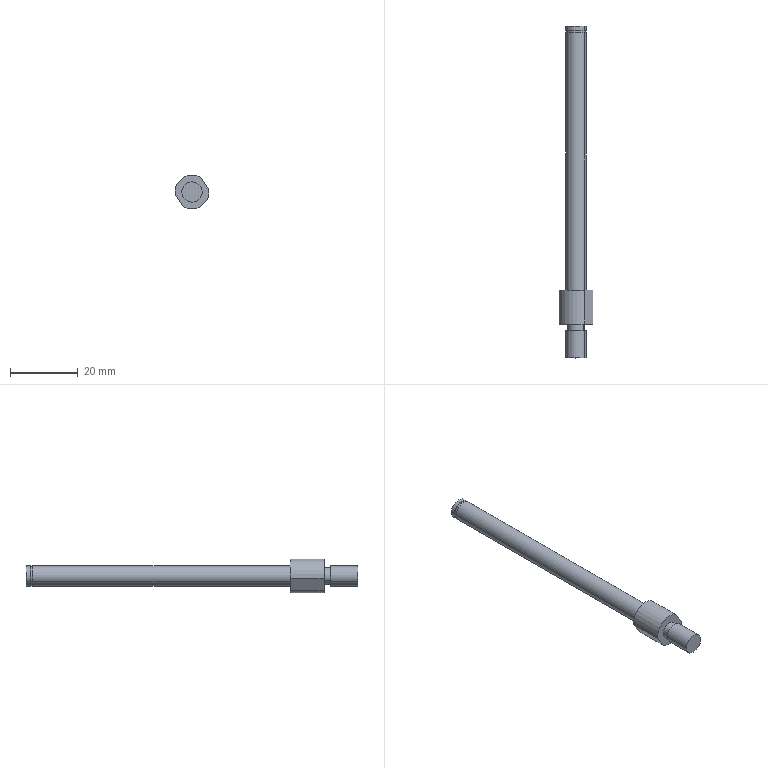Component | SolidWorks | JL001-03-06-4_JL001-03-06-001-1 | 1 solid | 21 faces | box 10 x 98 x 10 mm | volume 3224 mm3 | cylinder 12 | plane 9 | commonest cylinder face diameters 6 x6 5 x2 5.6 x2 10 x2
build123d program:
from build123d import *

# Parameters (mm, degrees)
SKETCH6_OUTSIDE_W   = 31.804
SKETCH6_OUTSIDE_H   = 31.804
SKETCH6_OUTSIDE_W_2 = 16.589
SKETCH6_OUTSIDE_H_2 = 9
CUT_EXTRUDE2_DEPTH  = 79.32


with BuildPart() as part:
    # Sketch1 → Revolve1 (revolve)
    with BuildSketch(Plane.XY, mode=Mode.PRIVATE) as revolve1_sk:
        Polygon((0, 98), (3, 98), (3, 96.8), (2.8, 96.8), (2.8, 96), (3, 96), (3, 20), (5, 20), (5, 10), (2.5, 10), (2.5, 8), (3, 8), (3, 0), (0, 0), align=None)
    revolve(revolve1_sk.sketch.rotate(Axis((0, 0, 0), (0, 1, 0)), 90), axis=Axis((0, 0, 0), (0, 1, 0)))

    # Sketch6 outside → Cut-Extrude2 (cut, through all)
    with BuildSketch(Plane(origin=(0, 20, 0), x_dir=(1, 0, 0), z_dir=(0, 1, 0))):
        Rectangle(SKETCH6_OUTSIDE_W, SKETCH6_OUTSIDE_H)
        Rectangle(SKETCH6_OUTSIDE_W_2, SKETCH6_OUTSIDE_H_2, mode=Mode.SUBTRACT)
    extrude(amount=-CUT_EXTRUDE2_DEPTH, mode=Mode.SUBTRACT)


solid = part.part

# Placed as in the assembly
solid = solid.moved(Location((-15, -47.5, 112.5), (-180, -56.842, -180)))
STEP:
#1=COLOUR_RGB('',0.7922,0.8196,0.9333);
#2=FILL_AREA_STYLE_COLOUR('',#1);
#3=FILL_AREA_STYLE('',(#2));
#4=SURFACE_STYLE_FILL_AREA(#3);
#5=SURFACE_SIDE_STYLE('',(#4));
#6=SURFACE_STYLE_USAGE(.BOTH.,#5);
#7=PRESENTATION_STYLE_ASSIGNMENT((#6));
#8=CARTESIAN_POINT('',(-0.4917,-1.555,4.494));
#9=VERTEX_POINT('',#8);
#10=CARTESIAN_POINT('',(-0.6894,-1.555,4.365));
#11=VERTEX_POINT('',#10);
#12=CARTESIAN_POINT('',(-0.5906,-1.555,4.429));
#13=DIRECTION('',(0.,-1.,0.));
#14=DIRECTION('',(0.8372,0.,0.5469));
#15=AXIS2_PLACEMENT_3D('',#12,#13,#14);
#16=CIRCLE('',#15,0.1181);
#17=EDGE_CURVE('',#9,#11,#16,.T.);
#18=ORIENTED_EDGE('',*,*,#17,.T.);
#19=CARTESIAN_POINT('',(-0.6894,-1.87,4.365));
#20=VERTEX_POINT('',#19);
#21=CARTESIAN_POINT('',(-0.6894,-1.87,4.365));
#22=DIRECTION('',(0.,-1.,0.));
#23=VECTOR('',#22,39.37);
#24=LINE('',#21,#23);
#25=EDGE_CURVE('',#11,#20,#24,.T.);
#26=ORIENTED_EDGE('',*,*,#25,.T.);
#27=CARTESIAN_POINT('',(-0.4917,-1.87,4.494));
#28=VERTEX_POINT('',#27);
#29=CARTESIAN_POINT('',(-0.5906,-1.87,4.429));
#30=DIRECTION('',(0.,-1.,0.));
#31=DIRECTION('',(0.8372,0.,0.5469));
#32=AXIS2_PLACEMENT_3D('',#29,#30,#31);
#33=CIRCLE('',#32,0.1181);
#34=EDGE_CURVE('',#28,#20,#33,.T.);
#35=ORIENTED_EDGE('',*,*,#34,.F.);
#36=CARTESIAN_POINT('',(-0.4917,-1.87,4.494));
#37=DIRECTION('',(0.,-1.,0.));
#38=VECTOR('',#37,39.37);
#39=LINE('',#36,#38);
#40=EDGE_CURVE('',#9,#28,#39,.T.);
#41=ORIENTED_EDGE('',*,*,#40,.F.);
#42=EDGE_LOOP('',(#18,#26,#35,#41));
#43=FACE_OUTER_BOUND('',#42,.T.);
#44=CARTESIAN_POINT('',(-0.5906,-1.87,4.429));
#45=DIRECTION('',(0.,-1.,0.));
#46=DIRECTION('',(0.8372,0.,0.5469));
#47=AXIS2_PLACEMENT_3D('',#44,#45,#46);
#48=CYLINDRICAL_SURFACE('',#47,0.1181);
#49=ADVANCED_FACE('',(#43),#48,.T.);
#50=CARTESIAN_POINT('',(-0.5082,-1.476,4.483));
#51=VERTEX_POINT('',#50);
#52=CARTESIAN_POINT('',(-0.6729,-1.476,4.375));
#53=VERTEX_POINT('',#52);
#54=CARTESIAN_POINT('',(-0.5906,-1.476,4.429));
#55=DIRECTION('',(0.,-1.,0.));
#56=DIRECTION('',(0.8372,0.,0.5469));
#57=AXIS2_PLACEMENT_3D('',#54,#55,#56);
#58=CIRCLE('',#57,0.09843);
#59=EDGE_CURVE('',#51,#53,#58,.T.);
#60=ORIENTED_EDGE('',*,*,#59,.T.);
#61=CARTESIAN_POINT('',(-0.6729,-1.555,4.375));
#62=VERTEX_POINT('',#61);
#63=CARTESIAN_POINT('',(-0.6729,-1.87,4.375));
#64=DIRECTION('',(0.,-1.,0.));
#65=VECTOR('',#64,39.37);
#66=LINE('',#63,#65);
#67=EDGE_CURVE('',#53,#62,#66,.T.);
#68=ORIENTED_EDGE('',*,*,#67,.T.);
#69=CARTESIAN_POINT('',(-0.5082,-1.555,4.483));
#70=VERTEX_POINT('',#69);
#71=CARTESIAN_POINT('',(-0.5906,-1.555,4.429));
#72=DIRECTION('',(0.,-1.,0.));
#73=DIRECTION('',(0.8372,0.,0.5469));
#74=AXIS2_PLACEMENT_3D('',#71,#72,#73);
#75=CIRCLE('',#74,0.09843);
#76=EDGE_CURVE('',#70,#62,#75,.T.);
#77=ORIENTED_EDGE('',*,*,#76,.F.);
#78=CARTESIAN_POINT('',(-0.5082,-1.87,4.483));
#79=DIRECTION('',(0.,-1.,0.));
#80=VECTOR('',#79,39.37);
#81=LINE('',#78,#80);
#82=EDGE_CURVE('',#51,#70,#81,.T.);
#83=ORIENTED_EDGE('',*,*,#82,.F.);
#84=EDGE_LOOP('',(#60,#68,#77,#83));
#85=FACE_OUTER_BOUND('',#84,.T.);
#86=CARTESIAN_POINT('',(-0.5906,-1.87,4.429));
#87=DIRECTION('',(0.,-1.,0.));
#88=DIRECTION('',(0.8372,0.,0.5469));
#89=AXIS2_PLACEMENT_3D('',#86,#87,#88);
#90=CYLINDRICAL_SURFACE('',#89,0.09843);
#91=ADVANCED_FACE('',(#85),#90,.T.);
#92=CARTESIAN_POINT('',(-0.4917,1.909,4.494));
#93=VERTEX_POINT('',#92);
#94=CARTESIAN_POINT('',(-0.6894,1.909,4.365));
#95=VERTEX_POINT('',#94);
#96=CARTESIAN_POINT('',(-0.5906,1.909,4.429));
#97=DIRECTION('',(0.,-1.,0.));
#98=DIRECTION('',(0.8372,0.,0.5469));
#99=AXIS2_PLACEMENT_3D('',#96,#97,#98);
#100=CIRCLE('',#99,0.1181);
#101=EDGE_CURVE('',#93,#95,#100,.T.);
#102=ORIENTED_EDGE('',*,*,#101,.T.);
#103=CARTESIAN_POINT('',(-0.6894,-1.083,4.365));
#104=VERTEX_POINT('',#103);
#105=CARTESIAN_POINT('',(-0.6894,-1.87,4.365));
#106=DIRECTION('',(0.,-1.,0.));
#107=VECTOR('',#106,39.37);
#108=LINE('',#105,#107);
#109=EDGE_CURVE('',#95,#104,#108,.T.);
#110=ORIENTED_EDGE('',*,*,#109,.T.);
#111=CARTESIAN_POINT('',(-0.4917,-1.083,4.494));
#112=VERTEX_POINT('',#111);
#113=CARTESIAN_POINT('',(-0.5906,-1.083,4.429));
#114=DIRECTION('',(0.,-1.,0.));
#115=DIRECTION('',(0.8372,0.,0.5469));
#116=AXIS2_PLACEMENT_3D('',#113,#114,#115);
#117=CIRCLE('',#116,0.1181);
#118=EDGE_CURVE('',#112,#104,#117,.T.);
#119=ORIENTED_EDGE('',*,*,#118,.F.);
#120=CARTESIAN_POINT('',(-0.4917,-1.87,4.494));
#121=DIRECTION('',(0.,-1.,0.));
#122=VECTOR('',#121,39.37);
#123=LINE('',#120,#122);
#124=EDGE_CURVE('',#93,#112,#123,.T.);
#125=ORIENTED_EDGE('',*,*,#124,.F.);
#126=EDGE_LOOP('',(#102,#110,#119,#125));
#127=FACE_OUTER_BOUND('',#126,.T.);
#128=CARTESIAN_POINT('',(-0.5906,-1.87,4.429));
#129=DIRECTION('',(0.,-1.,0.));
#130=DIRECTION('',(0.8372,0.,0.5469));
#131=AXIS2_PLACEMENT_3D('',#128,#129,#130);
#132=CYLINDRICAL_SURFACE('',#131,0.1181);
#133=ADVANCED_FACE('',(#127),#132,.T.);
#134=CARTESIAN_POINT('',(-0.4983,1.941,4.489));
#135=VERTEX_POINT('',#134);
#136=CARTESIAN_POINT('',(-0.6828,1.941,4.369));
#137=VERTEX_POINT('',#136);
#138=CARTESIAN_POINT('',(-0.5906,1.941,4.429));
#139=DIRECTION('',(0.,-1.,0.));
#140=DIRECTION('',(0.8372,0.,0.5469));
#141=AXIS2_PLACEMENT_3D('',#138,#139,#140);
#142=CIRCLE('',#141,0.1102);
#143=EDGE_CURVE('',#135,#137,#142,.T.);
#144=ORIENTED_EDGE('',*,*,#143,.T.);
#145=CARTESIAN_POINT('',(-0.6828,1.909,4.369));
#146=VERTEX_POINT('',#145);
#147=CARTESIAN_POINT('',(-0.6828,-1.87,4.369));
#148=DIRECTION('',(0.,-1.,0.));
#149=VECTOR('',#148,39.37);
#150=LINE('',#147,#149);
#151=EDGE_CURVE('',#137,#146,#150,.T.);
#152=ORIENTED_EDGE('',*,*,#151,.T.);
#153=CARTESIAN_POINT('',(-0.4983,1.909,4.489));
#154=VERTEX_POINT('',#153);
#155=CARTESIAN_POINT('',(-0.5906,1.909,4.429));
#156=DIRECTION('',(0.,-1.,0.));
#157=DIRECTION('',(0.8372,0.,0.5469));
#158=AXIS2_PLACEMENT_3D('',#155,#156,#157);
#159=CIRCLE('',#158,0.1102);
#160=EDGE_CURVE('',#154,#146,#159,.T.);
#161=ORIENTED_EDGE('',*,*,#160,.F.);
#162=CARTESIAN_POINT('',(-0.4983,-1.87,4.489));
#163=DIRECTION('',(0.,-1.,0.));
#164=VECTOR('',#163,39.37);
#165=LINE('',#162,#164);
#166=EDGE_CURVE('',#135,#154,#165,.T.);
#167=ORIENTED_EDGE('',*,*,#166,.F.);
#168=EDGE_LOOP('',(#144,#152,#161,#167));
#169=FACE_OUTER_BOUND('',#168,.T.);
#170=CARTESIAN_POINT('',(-0.5906,-1.87,4.429));
#171=DIRECTION('',(0.,-1.,0.));
#172=DIRECTION('',(0.8372,0.,0.5469));
#173=AXIS2_PLACEMENT_3D('',#170,#171,#172);
#174=CYLINDRICAL_SURFACE('',#173,0.1102);
#175=ADVANCED_FACE('',(#169),#174,.T.);
#176=CARTESIAN_POINT('',(-0.4917,1.988,4.494));
#177=VERTEX_POINT('',#176);
#178=CARTESIAN_POINT('',(-0.6894,1.988,4.365));
#179=VERTEX_POINT('',#178);
#180=CARTESIAN_POINT('',(-0.5906,1.988,4.429));
#181=DIRECTION('',(0.,-1.,0.));
#182=DIRECTION('',(0.8372,0.,0.5469));
#183=AXIS2_PLACEMENT_3D('',#180,#181,#182);
#184=CIRCLE('',#183,0.1181);
#185=EDGE_CURVE('',#177,#179,#184,.T.);
#186=ORIENTED_EDGE('',*,*,#185,.T.);
#187=CARTESIAN_POINT('',(-0.6894,1.941,4.365));
#188=VERTEX_POINT('',#187);
#189=CARTESIAN_POINT('',(-0.6894,-1.87,4.365));
#190=DIRECTION('',(0.,-1.,0.));
#191=VECTOR('',#190,39.37);
#192=LINE('',#189,#191);
#193=EDGE_CURVE('',#179,#188,#192,.T.);
#194=ORIENTED_EDGE('',*,*,#193,.T.);
#195=CARTESIAN_POINT('',(-0.4917,1.941,4.494));
#196=VERTEX_POINT('',#195);
#197=CARTESIAN_POINT('',(-0.5906,1.941,4.429));
#198=DIRECTION('',(0.,-1.,0.));
#199=DIRECTION('',(0.8372,0.,0.5469));
#200=AXIS2_PLACEMENT_3D('',#197,#198,#199);
#201=CIRCLE('',#200,0.1181);
#202=EDGE_CURVE('',#196,#188,#201,.T.);
#203=ORIENTED_EDGE('',*,*,#202,.F.);
#204=CARTESIAN_POINT('',(-0.4917,-1.87,4.494));
#205=DIRECTION('',(0.,-1.,0.));
#206=VECTOR('',#205,39.37);
#207=LINE('',#204,#206);
#208=EDGE_CURVE('',#177,#196,#207,.T.);
#209=ORIENTED_EDGE('',*,*,#208,.F.);
#210=EDGE_LOOP('',(#186,#194,#203,#209));
#211=FACE_OUTER_BOUND('',#210,.T.);
#212=CARTESIAN_POINT('',(-0.5906,-1.87,4.429));
#213=DIRECTION('',(0.,-1.,0.));
#214=DIRECTION('',(0.8372,0.,0.5469));
#215=AXIS2_PLACEMENT_3D('',#212,#213,#214);
#216=CYLINDRICAL_SURFACE('',#215,0.1181);
#217=ADVANCED_FACE('',(#211),#216,.T.);
#218=ORIENTED_EDGE('',*,*,#118,.T.);
#219=CARTESIAN_POINT('',(-0.5906,-1.083,4.429));
#220=DIRECTION('',(0.,-1.,0.));
#221=DIRECTION('',(0.8372,0.,0.5469));
#222=AXIS2_PLACEMENT_3D('',#219,#220,#221);
#223=CIRCLE('',#222,0.1181);
#224=EDGE_CURVE('',#104,#112,#223,.T.);
#225=ORIENTED_EDGE('',*,*,#224,.T.);
#226=EDGE_LOOP('',(#218,#225));
#227=FACE_BOUND('',#226,.T.);
#228=CARTESIAN_POINT('',(-0.6919,-1.083,4.26));
#229=VERTEX_POINT('',#228);
#230=CARTESIAN_POINT('',(-0.3953,-1.083,4.454));
#231=VERTEX_POINT('',#230);
#232=CARTESIAN_POINT('',(-0.5906,-1.083,4.429));
#233=DIRECTION('',(0.,-1.,0.));
#234=DIRECTION('',(0.8372,0.,0.5469));
#235=AXIS2_PLACEMENT_3D('',#232,#233,#234);
#236=CIRCLE('',#235,0.1969);
#237=EDGE_CURVE('',#229,#231,#236,.T.);
#238=ORIENTED_EDGE('',*,*,#237,.F.);
#239=CARTESIAN_POINT('',(-0.7858,-1.083,4.404));
#240=VERTEX_POINT('',#239);
#241=CARTESIAN_POINT('',(-0.5603,-1.083,4.059));
#242=DIRECTION('',(-0.5469,0.,0.8372));
#243=VECTOR('',#242,39.37);
#244=LINE('',#241,#243);
#245=EDGE_CURVE('',#229,#240,#244,.T.);
#246=ORIENTED_EDGE('',*,*,#245,.T.);
#247=CARTESIAN_POINT('',(-0.4892,-1.083,4.598));
#248=VERTEX_POINT('',#247);
#249=CARTESIAN_POINT('',(-0.5906,-1.083,4.429));
#250=DIRECTION('',(0.,-1.,0.));
#251=DIRECTION('',(0.8372,0.,0.5469));
#252=AXIS2_PLACEMENT_3D('',#249,#250,#251);
#253=CIRCLE('',#252,0.1969);
#254=EDGE_CURVE('',#248,#240,#253,.T.);
#255=ORIENTED_EDGE('',*,*,#254,.F.);
#256=CARTESIAN_POINT('',(-0.2636,-1.083,4.253));
#257=DIRECTION('',(0.5469,0.,-0.8372));
#258=VECTOR('',#257,39.37);
#259=LINE('',#256,#258);
#260=EDGE_CURVE('',#248,#231,#259,.T.);
#261=ORIENTED_EDGE('',*,*,#260,.T.);
#262=EDGE_LOOP('',(#238,#246,#255,#261));
#263=FACE_OUTER_BOUND('',#262,.T.);
#264=CARTESIAN_POINT('',(-0.6552,-1.083,4.528));
#265=DIRECTION('',(0.,1.,0.));
#266=DIRECTION('',(-0.8372,0.,-0.5469));
#267=AXIS2_PLACEMENT_3D('',#264,#265,#266);
#268=PLANE('',#267);
#269=ADVANCED_FACE('',(#227,#263),#268,.T.);
#270=CARTESIAN_POINT('',(-0.6919,-1.476,4.26));
#271=VERTEX_POINT('',#270);
#272=CARTESIAN_POINT('',(-0.3953,-1.476,4.454));
#273=VERTEX_POINT('',#272);
#274=CARTESIAN_POINT('',(-0.5906,-1.476,4.429));
#275=DIRECTION('',(0.,-1.,0.));
#276=DIRECTION('',(0.8372,0.,0.5469));
#277=AXIS2_PLACEMENT_3D('',#274,#275,#276);
#278=CIRCLE('',#277,0.1969);
#279=EDGE_CURVE('',#271,#273,#278,.T.);
#280=ORIENTED_EDGE('',*,*,#279,.F.);
#281=CARTESIAN_POINT('',(-0.6919,-1.87,4.26));
#282=DIRECTION('',(0.,1.,0.));
#283=VECTOR('',#282,39.37);
#284=LINE('',#281,#283);
#285=EDGE_CURVE('',#271,#229,#284,.T.);
#286=ORIENTED_EDGE('',*,*,#285,.T.);
#287=ORIENTED_EDGE('',*,*,#237,.T.);
#288=CARTESIAN_POINT('',(-0.3953,-1.87,4.454));
#289=DIRECTION('',(0.,-1.,0.));
#290=VECTOR('',#289,39.37);
#291=LINE('',#288,#290);
#292=EDGE_CURVE('',#231,#273,#291,.T.);
#293=ORIENTED_EDGE('',*,*,#292,.T.);
#294=EDGE_LOOP('',(#280,#286,#287,#293));
#295=FACE_OUTER_BOUND('',#294,.T.);
#296=CARTESIAN_POINT('',(-0.5906,-1.87,4.429));
#297=DIRECTION('',(0.,-1.,0.));
#298=DIRECTION('',(0.8372,0.,0.5469));
#299=AXIS2_PLACEMENT_3D('',#296,#297,#298);
#300=CYLINDRICAL_SURFACE('',#299,0.1969);
#301=ADVANCED_FACE('',(#295),#300,.T.);
#302=ORIENTED_EDGE('',*,*,#254,.T.);
#303=CARTESIAN_POINT('',(-0.7858,-1.476,4.404));
#304=VERTEX_POINT('',#303);
#305=CARTESIAN_POINT('',(-0.7858,-1.87,4.404));
#306=DIRECTION('',(0.,-1.,0.));
#307=VECTOR('',#306,39.37);
#308=LINE('',#305,#307);
#309=EDGE_CURVE('',#240,#304,#308,.T.);
#310=ORIENTED_EDGE('',*,*,#309,.T.);
#311=CARTESIAN_POINT('',(-0.4892,-1.476,4.598));
#312=VERTEX_POINT('',#311);
#313=CARTESIAN_POINT('',(-0.5906,-1.476,4.429));
#314=DIRECTION('',(0.,-1.,0.));
#315=DIRECTION('',(0.8372,0.,0.5469));
#316=AXIS2_PLACEMENT_3D('',#313,#314,#315);
#317=CIRCLE('',#316,0.1969);
#318=EDGE_CURVE('',#312,#304,#317,.T.);
#319=ORIENTED_EDGE('',*,*,#318,.F.);
#320=CARTESIAN_POINT('',(-0.4892,-1.87,4.598));
#321=DIRECTION('',(0.,1.,0.));
#322=VECTOR('',#321,39.37);
#323=LINE('',#320,#322);
#324=EDGE_CURVE('',#312,#248,#323,.T.);
#325=ORIENTED_EDGE('',*,*,#324,.T.);
#326=EDGE_LOOP('',(#302,#310,#319,#325));
#327=FACE_OUTER_BOUND('',#326,.T.);
#328=CARTESIAN_POINT('',(-0.5906,-1.87,4.429));
#329=DIRECTION('',(0.,-1.,0.));
#330=DIRECTION('',(0.8372,0.,0.5469));
#331=AXIS2_PLACEMENT_3D('',#328,#329,#330);
#332=CYLINDRICAL_SURFACE('',#331,0.1969);
#333=ADVANCED_FACE('',(#327),#332,.T.);
#334=ORIENTED_EDGE('',*,*,#59,.F.);
#335=CARTESIAN_POINT('',(-0.5906,-1.476,4.429));
#336=DIRECTION('',(0.,-1.,0.));
#337=DIRECTION('',(0.8372,0.,0.5469));
#338=AXIS2_PLACEMENT_3D('',#335,#336,#337);
#339=CIRCLE('',#338,0.09843);
#340=EDGE_CURVE('',#53,#51,#339,.T.);
#341=ORIENTED_EDGE('',*,*,#340,.F.);
#342=EDGE_LOOP('',(#334,#341));
#343=FACE_BOUND('',#342,.T.);
#344=ORIENTED_EDGE('',*,*,#318,.T.);
#345=CARTESIAN_POINT('',(-0.8465,-1.476,4.497));
#346=DIRECTION('',(0.5469,0.,-0.8372));
#347=VECTOR('',#346,39.37);
#348=LINE('',#345,#347);
#349=EDGE_CURVE('',#304,#271,#348,.T.);
#350=ORIENTED_EDGE('',*,*,#349,.T.);
#351=ORIENTED_EDGE('',*,*,#279,.T.);
#352=CARTESIAN_POINT('',(-0.5499,-1.476,4.691));
#353=DIRECTION('',(-0.5469,0.,0.8372));
#354=VECTOR('',#353,39.37);
#355=LINE('',#352,#354);
#356=EDGE_CURVE('',#273,#312,#355,.T.);
#357=ORIENTED_EDGE('',*,*,#356,.T.);
#358=EDGE_LOOP('',(#344,#350,#351,#357));
#359=FACE_OUTER_BOUND('',#358,.T.);
#360=CARTESIAN_POINT('',(-0.6982,-1.476,4.594));
#361=DIRECTION('',(0.,-1.,0.));
#362=DIRECTION('',(0.8372,0.,0.5469));
#363=AXIS2_PLACEMENT_3D('',#360,#361,#362);
#364=PLANE('',#363);
#365=ADVANCED_FACE('',(#343,#359),#364,.T.);
#366=ORIENTED_EDGE('',*,*,#185,.F.);
#367=CARTESIAN_POINT('',(-0.5906,1.988,4.429));
#368=DIRECTION('',(0.,-1.,0.));
#369=DIRECTION('',(0.8372,0.,0.5469));
#370=AXIS2_PLACEMENT_3D('',#367,#368,#369);
#371=CIRCLE('',#370,0.1181);
#372=EDGE_CURVE('',#179,#177,#371,.T.);
#373=ORIENTED_EDGE('',*,*,#372,.F.);
#374=EDGE_LOOP('',(#366,#373));
#375=FACE_OUTER_BOUND('',#374,.T.);
#376=CARTESIAN_POINT('',(-0.5906,1.988,4.429));
#377=DIRECTION('',(0.,1.,0.));
#378=DIRECTION('',(-0.8372,0.,-0.5469));
#379=AXIS2_PLACEMENT_3D('',#376,#377,#378);
#380=PLANE('',#379);
#381=ADVANCED_FACE('',(#375),#380,.T.);
#382=ORIENTED_EDGE('',*,*,#193,.F.);
#383=ORIENTED_EDGE('',*,*,#372,.T.);
#384=ORIENTED_EDGE('',*,*,#208,.T.);
#385=CARTESIAN_POINT('',(-0.5906,1.941,4.429));
#386=DIRECTION('',(0.,-1.,0.));
#387=DIRECTION('',(0.8372,0.,0.5469));
#388=AXIS2_PLACEMENT_3D('',#385,#386,#387);
#389=CIRCLE('',#388,0.1181);
#390=EDGE_CURVE('',#188,#196,#389,.T.);
#391=ORIENTED_EDGE('',*,*,#390,.F.);
#392=EDGE_LOOP('',(#382,#383,#384,#391));
#393=FACE_OUTER_BOUND('',#392,.T.);
#394=CARTESIAN_POINT('',(-0.5906,-1.87,4.429));
#395=DIRECTION('',(0.,-1.,0.));
#396=DIRECTION('',(0.8372,0.,0.5469));
#397=AXIS2_PLACEMENT_3D('',#394,#395,#396);
#398=CYLINDRICAL_SURFACE('',#397,0.1181);
#399=ADVANCED_FACE('',(#393),#398,.T.);
#400=ORIENTED_EDGE('',*,*,#202,.T.);
#401=ORIENTED_EDGE('',*,*,#390,.T.);
#402=EDGE_LOOP('',(#400,#401));
#403=FACE_OUTER_BOUND('',#402,.T.);
#404=ORIENTED_EDGE('',*,*,#143,.F.);
#405=CARTESIAN_POINT('',(-0.5906,1.941,4.429));
#406=DIRECTION('',(0.,-1.,0.));
#407=DIRECTION('',(0.8372,0.,0.5469));
#408=AXIS2_PLACEMENT_3D('',#405,#406,#407);
#409=CIRCLE('',#408,0.1102);
#410=EDGE_CURVE('',#137,#135,#409,.T.);
#411=ORIENTED_EDGE('',*,*,#410,.F.);
#412=EDGE_LOOP('',(#404,#411));
#413=FACE_BOUND('',#412,.T.);
#414=CARTESIAN_POINT('',(-0.6552,1.941,4.528));
#415=DIRECTION('',(0.,-1.,0.));
#416=DIRECTION('',(0.8372,0.,0.5469));
#417=AXIS2_PLACEMENT_3D('',#414,#415,#416);
#418=PLANE('',#417);
#419=ADVANCED_FACE('',(#403,#413),#418,.T.);
#420=ORIENTED_EDGE('',*,*,#151,.F.);
#421=ORIENTED_EDGE('',*,*,#410,.T.);
#422=ORIENTED_EDGE('',*,*,#166,.T.);
#423=CARTESIAN_POINT('',(-0.5906,1.909,4.429));
#424=DIRECTION('',(0.,-1.,0.));
#425=DIRECTION('',(0.8372,0.,0.5469));
#426=AXIS2_PLACEMENT_3D('',#423,#424,#425);
#427=CIRCLE('',#426,0.1102);
#428=EDGE_CURVE('',#146,#154,#427,.T.);
#429=ORIENTED_EDGE('',*,*,#428,.F.);
#430=EDGE_LOOP('',(#420,#421,#422,#429));
#431=FACE_OUTER_BOUND('',#430,.T.);
#432=CARTESIAN_POINT('',(-0.5906,-1.87,4.429));
#433=DIRECTION('',(0.,-1.,0.));
#434=DIRECTION('',(0.8372,0.,0.5469));
#435=AXIS2_PLACEMENT_3D('',#432,#433,#434);
#436=CYLINDRICAL_SURFACE('',#435,0.1102);
#437=ADVANCED_FACE('',(#431),#436,.T.);
#438=ORIENTED_EDGE('',*,*,#160,.T.);
#439=ORIENTED_EDGE('',*,*,#428,.T.);
#440=EDGE_LOOP('',(#438,#439));
#441=FACE_BOUND('',#440,.T.);
#442=ORIENTED_EDGE('',*,*,#101,.F.);
#443=CARTESIAN_POINT('',(-0.5906,1.909,4.429));
#444=DIRECTION('',(0.,-1.,0.));
#445=DIRECTION('',(0.8372,0.,0.5469));
#446=AXIS2_PLACEMENT_3D('',#443,#444,#445);
#447=CIRCLE('',#446,0.1181);
#448=EDGE_CURVE('',#95,#93,#447,.T.);
#449=ORIENTED_EDGE('',*,*,#448,.F.);
#450=EDGE_LOOP('',(#442,#449));
#451=FACE_OUTER_BOUND('',#450,.T.);
#452=CARTESIAN_POINT('',(-0.6508,1.909,4.521));
#453=DIRECTION('',(0.,1.,0.));
#454=DIRECTION('',(-0.8372,0.,-0.5469));
#455=AXIS2_PLACEMENT_3D('',#452,#453,#454);
#456=PLANE('',#455);
#457=ADVANCED_FACE('',(#441,#451),#456,.T.);
#458=ORIENTED_EDGE('',*,*,#109,.F.);
#459=ORIENTED_EDGE('',*,*,#448,.T.);
#460=ORIENTED_EDGE('',*,*,#124,.T.);
#461=ORIENTED_EDGE('',*,*,#224,.F.);
#462=EDGE_LOOP('',(#458,#459,#460,#461));
#463=FACE_OUTER_BOUND('',#462,.T.);
#464=CARTESIAN_POINT('',(-0.5906,-1.87,4.429));
#465=DIRECTION('',(0.,-1.,0.));
#466=DIRECTION('',(0.8372,0.,0.5469));
#467=AXIS2_PLACEMENT_3D('',#464,#465,#466);
#468=CYLINDRICAL_SURFACE('',#467,0.1181);
#469=ADVANCED_FACE('',(#463),#468,.T.);
#470=ORIENTED_EDGE('',*,*,#67,.F.);
#471=ORIENTED_EDGE('',*,*,#340,.T.);
#472=ORIENTED_EDGE('',*,*,#82,.T.);
#473=CARTESIAN_POINT('',(-0.5906,-1.555,4.429));
#474=DIRECTION('',(0.,-1.,0.));
#475=DIRECTION('',(0.8372,0.,0.5469));
#476=AXIS2_PLACEMENT_3D('',#473,#474,#475);
#477=CIRCLE('',#476,0.09843);
#478=EDGE_CURVE('',#62,#70,#477,.T.);
#479=ORIENTED_EDGE('',*,*,#478,.F.);
#480=EDGE_LOOP('',(#470,#471,#472,#479));
#481=FACE_OUTER_BOUND('',#480,.T.);
#482=CARTESIAN_POINT('',(-0.5906,-1.87,4.429));
#483=DIRECTION('',(0.,-1.,0.));
#484=DIRECTION('',(0.8372,0.,0.5469));
#485=AXIS2_PLACEMENT_3D('',#482,#483,#484);
#486=CYLINDRICAL_SURFACE('',#485,0.09843);
#487=ADVANCED_FACE('',(#481),#486,.T.);
#488=ORIENTED_EDGE('',*,*,#76,.T.);
#489=ORIENTED_EDGE('',*,*,#478,.T.);
#490=EDGE_LOOP('',(#488,#489));
#491=FACE_BOUND('',#490,.T.);
#492=ORIENTED_EDGE('',*,*,#17,.F.);
#493=CARTESIAN_POINT('',(-0.5906,-1.555,4.429));
#494=DIRECTION('',(0.,-1.,0.));
#495=DIRECTION('',(0.8372,0.,0.5469));
#496=AXIS2_PLACEMENT_3D('',#493,#494,#495);
#497=CIRCLE('',#496,0.1181);
#498=EDGE_CURVE('',#11,#9,#497,.T.);
#499=ORIENTED_EDGE('',*,*,#498,.F.);
#500=EDGE_LOOP('',(#492,#499));
#501=FACE_OUTER_BOUND('',#500,.T.);
#502=CARTESIAN_POINT('',(-0.6444,-1.555,4.512));
#503=DIRECTION('',(0.,1.,0.));
#504=DIRECTION('',(-0.8372,0.,-0.5469));
#505=AXIS2_PLACEMENT_3D('',#502,#503,#504);
#506=PLANE('',#505);
#507=ADVANCED_FACE('',(#491,#501),#506,.T.);
#508=ORIENTED_EDGE('',*,*,#25,.F.);
#509=ORIENTED_EDGE('',*,*,#498,.T.);
#510=ORIENTED_EDGE('',*,*,#40,.T.);
#511=CARTESIAN_POINT('',(-0.5906,-1.87,4.429));
#512=DIRECTION('',(0.,-1.,0.));
#513=DIRECTION('',(0.8372,0.,0.5469));
#514=AXIS2_PLACEMENT_3D('',#511,#512,#513);
#515=CIRCLE('',#514,0.1181);
#516=EDGE_CURVE('',#20,#28,#515,.T.);
#517=ORIENTED_EDGE('',*,*,#516,.F.);
#518=EDGE_LOOP('',(#508,#509,#510,#517));
#519=FACE_OUTER_BOUND('',#518,.T.);
#520=CARTESIAN_POINT('',(-0.5906,-1.87,4.429));
#521=DIRECTION('',(0.,-1.,0.));
#522=DIRECTION('',(0.8372,0.,0.5469));
#523=AXIS2_PLACEMENT_3D('',#520,#521,#522);
#524=CYLINDRICAL_SURFACE('',#523,0.1181);
#525=ADVANCED_FACE('',(#519),#524,.T.);
#526=ORIENTED_EDGE('',*,*,#34,.T.);
#527=ORIENTED_EDGE('',*,*,#516,.T.);
#528=EDGE_LOOP('',(#526,#527));
#529=FACE_OUTER_BOUND('',#528,.T.);
#530=CARTESIAN_POINT('',(-0.6552,-1.87,4.528));
#531=DIRECTION('',(0.,-1.,0.));
#532=DIRECTION('',(0.8372,0.,0.5469));
#533=AXIS2_PLACEMENT_3D('',#530,#531,#532);
#534=PLANE('',#533);
#535=ADVANCED_FACE('',(#529),#534,.T.);
#536=ORIENTED_EDGE('',*,*,#356,.F.);
#537=ORIENTED_EDGE('',*,*,#292,.F.);
#538=ORIENTED_EDGE('',*,*,#260,.F.);
#539=ORIENTED_EDGE('',*,*,#324,.F.);
#540=EDGE_LOOP('',(#536,#537,#538,#539));
#541=FACE_OUTER_BOUND('',#540,.T.);
#542=CARTESIAN_POINT('',(-0.2636,-1.87,4.253));
#543=DIRECTION('',(0.8372,0.,0.5469));
#544=DIRECTION('',(0.5469,0.,-0.8372));
#545=AXIS2_PLACEMENT_3D('',#542,#543,#544);
#546=PLANE('',#545);
#547=ADVANCED_FACE('',(#541),#546,.T.);
#548=ORIENTED_EDGE('',*,*,#349,.F.);
#549=ORIENTED_EDGE('',*,*,#309,.F.);
#550=ORIENTED_EDGE('',*,*,#245,.F.);
#551=ORIENTED_EDGE('',*,*,#285,.F.);
#552=EDGE_LOOP('',(#548,#549,#550,#551));
#553=FACE_OUTER_BOUND('',#552,.T.);
#554=CARTESIAN_POINT('',(-0.5603,-1.87,4.059));
#555=DIRECTION('',(-0.8372,0.,-0.5469));
#556=DIRECTION('',(-0.5469,0.,0.8372));
#557=AXIS2_PLACEMENT_3D('',#554,#555,#556);
#558=PLANE('',#557);
#559=ADVANCED_FACE('',(#553),#558,.T.);
#560=CLOSED_SHELL('',(#49,#91,#133,#175,#217,#269,#301,#333,#365,#381,#399,#419,#437,#457,#469,#487,#507,#525,#535,#547,#559));
#561=MANIFOLD_SOLID_BREP('',#560);
#562=STYLED_ITEM('',(#7),#561);
#563=PRESENTATION_LAYER_ASSIGNMENT('','',(#562));
#564=(LENGTH_UNIT()NAMED_UNIT(*)SI_UNIT($,.METRE.));
#565=LENGTH_MEASURE_WITH_UNIT(LENGTH_MEASURE(0.0254),#564);
#566=DIMENSIONAL_EXPONENTS(1.,0.,0.,0.,0.,0.,0.);
#567=(CONVERSION_BASED_UNIT('',#565)LENGTH_UNIT()NAMED_UNIT(#566));
#568=UNCERTAINTY_MEASURE_WITH_UNIT(LENGTH_MEASURE(0.00001),#567,'','');
#569=(NAMED_UNIT(*)PLANE_ANGLE_UNIT()SI_UNIT($,.RADIAN.));
#570=(NAMED_UNIT(*)SI_UNIT($,.STERADIAN.)SOLID_ANGLE_UNIT());
#571=(GEOMETRIC_REPRESENTATION_CONTEXT(3)GLOBAL_UNCERTAINTY_ASSIGNED_CONTEXT((#568))GLOBAL_UNIT_ASSIGNED_CONTEXT((#567,#569,#570))REPRESENTATION_CONTEXT('',''));
#572=MECHANICAL_DESIGN_GEOMETRIC_PRESENTATION_REPRESENTATION('',(#562),#571);
#573=CARTESIAN_POINT('',(0.,0.,0.));
#574=DIRECTION('',(0.,0.,1.));
#575=DIRECTION('',(1.,0.,0.));
#576=AXIS2_PLACEMENT_3D('',#573,#574,#575);
#577=(LENGTH_UNIT()NAMED_UNIT(*)SI_UNIT($,.METRE.));
#578=LENGTH_MEASURE_WITH_UNIT(LENGTH_MEASURE(0.0254),#577);
#579=DIMENSIONAL_EXPONENTS(1.,0.,0.,0.,0.,0.,0.);
#580=(CONVERSION_BASED_UNIT('',#578)LENGTH_UNIT()NAMED_UNIT(#579));
#581=UNCERTAINTY_MEASURE_WITH_UNIT(LENGTH_MEASURE(0.00001),#580,'','');
#582=(NAMED_UNIT(*)PLANE_ANGLE_UNIT()SI_UNIT($,.RADIAN.));
#583=(NAMED_UNIT(*)SI_UNIT($,.STERADIAN.)SOLID_ANGLE_UNIT());
#584=(GEOMETRIC_REPRESENTATION_CONTEXT(3)GLOBAL_UNCERTAINTY_ASSIGNED_CONTEXT((#581))GLOBAL_UNIT_ASSIGNED_CONTEXT((#580,#582,#583))REPRESENTATION_CONTEXT('',''));
#585=ADVANCED_BREP_SHAPE_REPRESENTATION('',(#561,#576),#584);